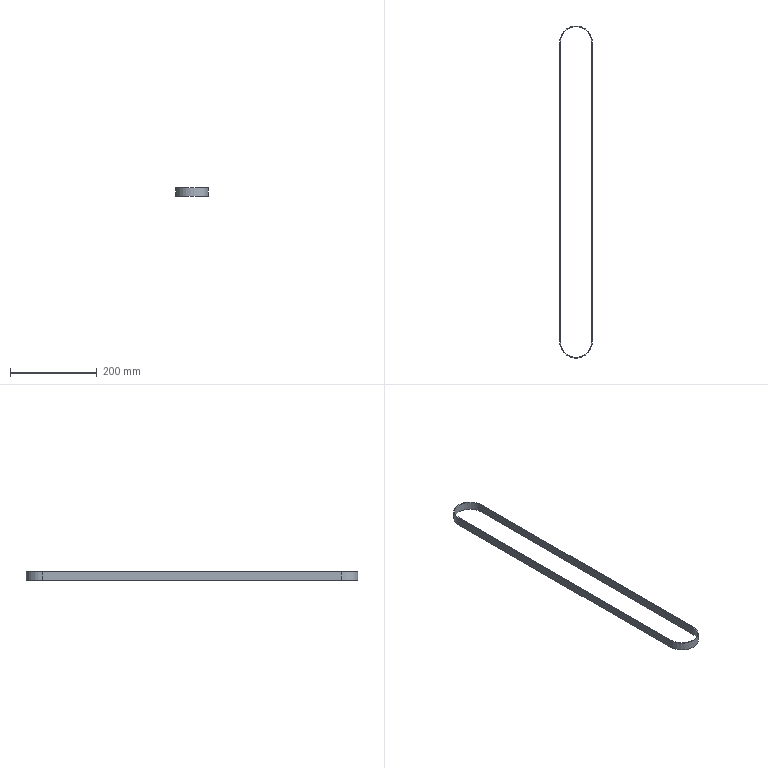Component | SolidWorks | tongbudai-1 | 1 solid | 10 faces | box 75.4 x 765.4 x 19 mm | volume 61203 mm3 | plane 6 | cylinder 4 | commonest cylinder face diameters 75.4 x2 71.4 x2
build123d program:
from build123d import *

# Parameters (mm, degrees)
EXTRUDE_THIN1_DEPTH = 9.5


with BuildPart() as part:
    # Sketch1 → Extrude-Thin1 (new, symmetric)
    with BuildSketch(Plane.XY):
        with BuildLine():
            Line((-37.7, -345), (-37.7, 345))
            ThreePointArc((-37.7, 345), (0, 382.7), (37.7, 345))
            Line((37.7, 345), (37.7, -345))
            ThreePointArc((37.7, -345), (0, -382.7), (-37.7, -345))
        make_face()
        with BuildLine():
            Line((-35.7, -345), (-35.7, 345))
            ThreePointArc((-35.7, 345), (0, 380.7), (35.7, 345))
            Line((35.7, 345), (35.7, -345))
            ThreePointArc((35.7, -345), (0, -380.7), (-35.7, -345))
        make_face(mode=Mode.SUBTRACT)
    extrude(amount=EXTRUDE_THIN1_DEPTH, both=True)


solid = part.part

# Placed as in the assembly
solid = solid.moved(Location((-25.633, -29.591, 38.5), (0, 0, 0)))
STEP:
#1=COLOUR_RGB('',0.7922,0.8196,0.9333);
#2=FILL_AREA_STYLE_COLOUR('',#1);
#3=FILL_AREA_STYLE('',(#2));
#4=SURFACE_STYLE_FILL_AREA(#3);
#5=SURFACE_SIDE_STYLE('',(#4));
#6=SURFACE_STYLE_USAGE(.BOTH.,#5);
#7=PRESENTATION_STYLE_ASSIGNMENT((#6));
#8=CARTESIAN_POINT('',(0.4751,12.418,1.89));
#9=VERTEX_POINT('',#8);
#10=CARTESIAN_POINT('',(-2.493,12.418,1.89));
#11=VERTEX_POINT('',#10);
#12=CARTESIAN_POINT('',(-1.009,12.418,1.89));
#13=DIRECTION('',(0.,0.,1.));
#14=DIRECTION('',(1.,0.,0.));
#15=AXIS2_PLACEMENT_3D('',#12,#13,#14);
#16=CIRCLE('',#15,1.484);
#17=EDGE_CURVE('',#9,#11,#16,.T.);
#18=ORIENTED_EDGE('',*,*,#17,.T.);
#19=CARTESIAN_POINT('',(-2.493,-14.748,1.89));
#20=VERTEX_POINT('',#19);
#21=CARTESIAN_POINT('',(-2.493,12.418,1.89));
#22=DIRECTION('',(0.,-1.,0.));
#23=VECTOR('',#22,39.37);
#24=LINE('',#21,#23);
#25=EDGE_CURVE('',#11,#20,#24,.T.);
#26=ORIENTED_EDGE('',*,*,#25,.T.);
#27=CARTESIAN_POINT('',(0.4751,-14.748,1.89));
#28=VERTEX_POINT('',#27);
#29=CARTESIAN_POINT('',(-1.009,-14.748,1.89));
#30=DIRECTION('',(0.,0.,1.));
#31=DIRECTION('',(1.,0.,0.));
#32=AXIS2_PLACEMENT_3D('',#29,#30,#31);
#33=CIRCLE('',#32,1.484);
#34=EDGE_CURVE('',#20,#28,#33,.T.);
#35=ORIENTED_EDGE('',*,*,#34,.T.);
#36=CARTESIAN_POINT('',(0.4751,12.418,1.89));
#37=DIRECTION('',(0.,1.,0.));
#38=VECTOR('',#37,39.37);
#39=LINE('',#36,#38);
#40=EDGE_CURVE('',#28,#9,#39,.T.);
#41=ORIENTED_EDGE('',*,*,#40,.T.);
#42=EDGE_LOOP('',(#18,#26,#35,#41));
#43=FACE_OUTER_BOUND('',#42,.T.);
#44=CARTESIAN_POINT('',(-2.415,12.418,1.89));
#45=VERTEX_POINT('',#44);
#46=CARTESIAN_POINT('',(-2.415,-14.748,1.89));
#47=VERTEX_POINT('',#46);
#48=CARTESIAN_POINT('',(-2.415,12.418,1.89));
#49=DIRECTION('',(0.,-1.,0.));
#50=VECTOR('',#49,39.37);
#51=LINE('',#48,#50);
#52=EDGE_CURVE('',#45,#47,#51,.T.);
#53=ORIENTED_EDGE('',*,*,#52,.F.);
#54=CARTESIAN_POINT('',(0.3963,12.418,1.89));
#55=VERTEX_POINT('',#54);
#56=CARTESIAN_POINT('',(-1.009,12.418,1.89));
#57=DIRECTION('',(0.,0.,1.));
#58=DIRECTION('',(1.,0.,0.));
#59=AXIS2_PLACEMENT_3D('',#56,#57,#58);
#60=CIRCLE('',#59,1.406);
#61=EDGE_CURVE('',#55,#45,#60,.T.);
#62=ORIENTED_EDGE('',*,*,#61,.F.);
#63=CARTESIAN_POINT('',(0.3963,-14.748,1.89));
#64=VERTEX_POINT('',#63);
#65=CARTESIAN_POINT('',(0.3963,12.418,1.89));
#66=DIRECTION('',(0.,1.,0.));
#67=VECTOR('',#66,39.37);
#68=LINE('',#65,#67);
#69=EDGE_CURVE('',#64,#55,#68,.T.);
#70=ORIENTED_EDGE('',*,*,#69,.F.);
#71=CARTESIAN_POINT('',(-1.009,-14.748,1.89));
#72=DIRECTION('',(0.,0.,1.));
#73=DIRECTION('',(1.,0.,0.));
#74=AXIS2_PLACEMENT_3D('',#71,#72,#73);
#75=CIRCLE('',#74,1.406);
#76=EDGE_CURVE('',#47,#64,#75,.T.);
#77=ORIENTED_EDGE('',*,*,#76,.F.);
#78=EDGE_LOOP('',(#53,#62,#70,#77));
#79=FACE_BOUND('',#78,.T.);
#80=CARTESIAN_POINT('',(-1.009,12.418,1.89));
#81=DIRECTION('',(0.,0.,1.));
#82=DIRECTION('',(1.,0.,0.));
#83=AXIS2_PLACEMENT_3D('',#80,#81,#82);
#84=PLANE('',#83);
#85=ADVANCED_FACE('',(#43,#79),#84,.T.);
#86=CARTESIAN_POINT('',(0.4751,12.418,1.142));
#87=VERTEX_POINT('',#86);
#88=CARTESIAN_POINT('',(-2.493,12.418,1.142));
#89=VERTEX_POINT('',#88);
#90=CARTESIAN_POINT('',(-1.009,12.418,1.142));
#91=DIRECTION('',(0.,0.,1.));
#92=DIRECTION('',(1.,0.,0.));
#93=AXIS2_PLACEMENT_3D('',#90,#91,#92);
#94=CIRCLE('',#93,1.484);
#95=EDGE_CURVE('',#87,#89,#94,.T.);
#96=ORIENTED_EDGE('',*,*,#95,.F.);
#97=CARTESIAN_POINT('',(0.4751,-14.748,1.142));
#98=VERTEX_POINT('',#97);
#99=CARTESIAN_POINT('',(0.4751,12.418,1.142));
#100=DIRECTION('',(0.,1.,0.));
#101=VECTOR('',#100,39.37);
#102=LINE('',#99,#101);
#103=EDGE_CURVE('',#98,#87,#102,.T.);
#104=ORIENTED_EDGE('',*,*,#103,.F.);
#105=CARTESIAN_POINT('',(-2.493,-14.748,1.142));
#106=VERTEX_POINT('',#105);
#107=CARTESIAN_POINT('',(-1.009,-14.748,1.142));
#108=DIRECTION('',(0.,0.,1.));
#109=DIRECTION('',(1.,0.,0.));
#110=AXIS2_PLACEMENT_3D('',#107,#108,#109);
#111=CIRCLE('',#110,1.484);
#112=EDGE_CURVE('',#106,#98,#111,.T.);
#113=ORIENTED_EDGE('',*,*,#112,.F.);
#114=CARTESIAN_POINT('',(-2.493,12.418,1.142));
#115=DIRECTION('',(0.,-1.,0.));
#116=VECTOR('',#115,39.37);
#117=LINE('',#114,#116);
#118=EDGE_CURVE('',#89,#106,#117,.T.);
#119=ORIENTED_EDGE('',*,*,#118,.F.);
#120=EDGE_LOOP('',(#96,#104,#113,#119));
#121=FACE_OUTER_BOUND('',#120,.T.);
#122=CARTESIAN_POINT('',(0.3963,12.418,1.142));
#123=VERTEX_POINT('',#122);
#124=CARTESIAN_POINT('',(-2.415,12.418,1.142));
#125=VERTEX_POINT('',#124);
#126=CARTESIAN_POINT('',(-1.009,12.418,1.142));
#127=DIRECTION('',(0.,0.,1.));
#128=DIRECTION('',(1.,0.,0.));
#129=AXIS2_PLACEMENT_3D('',#126,#127,#128);
#130=CIRCLE('',#129,1.406);
#131=EDGE_CURVE('',#123,#125,#130,.T.);
#132=ORIENTED_EDGE('',*,*,#131,.T.);
#133=CARTESIAN_POINT('',(-2.415,-14.748,1.142));
#134=VERTEX_POINT('',#133);
#135=CARTESIAN_POINT('',(-2.415,12.418,1.142));
#136=DIRECTION('',(0.,-1.,0.));
#137=VECTOR('',#136,39.37);
#138=LINE('',#135,#137);
#139=EDGE_CURVE('',#125,#134,#138,.T.);
#140=ORIENTED_EDGE('',*,*,#139,.T.);
#141=CARTESIAN_POINT('',(0.3963,-14.748,1.142));
#142=VERTEX_POINT('',#141);
#143=CARTESIAN_POINT('',(-1.009,-14.748,1.142));
#144=DIRECTION('',(0.,0.,1.));
#145=DIRECTION('',(1.,0.,0.));
#146=AXIS2_PLACEMENT_3D('',#143,#144,#145);
#147=CIRCLE('',#146,1.406);
#148=EDGE_CURVE('',#134,#142,#147,.T.);
#149=ORIENTED_EDGE('',*,*,#148,.T.);
#150=CARTESIAN_POINT('',(0.3963,12.418,1.142));
#151=DIRECTION('',(0.,1.,0.));
#152=VECTOR('',#151,39.37);
#153=LINE('',#150,#152);
#154=EDGE_CURVE('',#142,#123,#153,.T.);
#155=ORIENTED_EDGE('',*,*,#154,.T.);
#156=EDGE_LOOP('',(#132,#140,#149,#155));
#157=FACE_BOUND('',#156,.T.);
#158=CARTESIAN_POINT('',(-1.009,12.418,1.142));
#159=DIRECTION('',(0.,0.,1.));
#160=DIRECTION('',(1.,0.,0.));
#161=AXIS2_PLACEMENT_3D('',#158,#159,#160);
#162=PLANE('',#161);
#163=ADVANCED_FACE('',(#121,#157),#162,.F.);
#164=ORIENTED_EDGE('',*,*,#95,.T.);
#165=CARTESIAN_POINT('',(-2.493,12.418,1.89));
#166=DIRECTION('',(0.,0.,-1.));
#167=VECTOR('',#166,39.37);
#168=LINE('',#165,#167);
#169=EDGE_CURVE('',#11,#89,#168,.T.);
#170=ORIENTED_EDGE('',*,*,#169,.F.);
#171=ORIENTED_EDGE('',*,*,#17,.F.);
#172=CARTESIAN_POINT('',(0.4751,12.418,1.89));
#173=DIRECTION('',(0.,0.,-1.));
#174=VECTOR('',#173,39.37);
#175=LINE('',#172,#174);
#176=EDGE_CURVE('',#9,#87,#175,.T.);
#177=ORIENTED_EDGE('',*,*,#176,.T.);
#178=EDGE_LOOP('',(#164,#170,#171,#177));
#179=FACE_OUTER_BOUND('',#178,.T.);
#180=CARTESIAN_POINT('',(-1.009,12.418,1.89));
#181=DIRECTION('',(0.,0.,-1.));
#182=DIRECTION('',(-1.,0.,0.));
#183=AXIS2_PLACEMENT_3D('',#180,#181,#182);
#184=CYLINDRICAL_SURFACE('',#183,1.484);
#185=ADVANCED_FACE('',(#179),#184,.T.);
#186=ORIENTED_EDGE('',*,*,#118,.T.);
#187=CARTESIAN_POINT('',(-2.493,-14.748,1.89));
#188=DIRECTION('',(0.,0.,-1.));
#189=VECTOR('',#188,39.37);
#190=LINE('',#187,#189);
#191=EDGE_CURVE('',#20,#106,#190,.T.);
#192=ORIENTED_EDGE('',*,*,#191,.F.);
#193=ORIENTED_EDGE('',*,*,#25,.F.);
#194=ORIENTED_EDGE('',*,*,#169,.T.);
#195=EDGE_LOOP('',(#186,#192,#193,#194));
#196=FACE_OUTER_BOUND('',#195,.T.);
#197=CARTESIAN_POINT('',(-2.493,12.418,1.89));
#198=DIRECTION('',(1.,0.,0.));
#199=DIRECTION('',(0.,0.,-1.));
#200=AXIS2_PLACEMENT_3D('',#197,#198,#199);
#201=PLANE('',#200);
#202=ADVANCED_FACE('',(#196),#201,.F.);
#203=ORIENTED_EDGE('',*,*,#112,.T.);
#204=CARTESIAN_POINT('',(0.4751,-14.748,1.89));
#205=DIRECTION('',(0.,0.,-1.));
#206=VECTOR('',#205,39.37);
#207=LINE('',#204,#206);
#208=EDGE_CURVE('',#28,#98,#207,.T.);
#209=ORIENTED_EDGE('',*,*,#208,.F.);
#210=ORIENTED_EDGE('',*,*,#34,.F.);
#211=ORIENTED_EDGE('',*,*,#191,.T.);
#212=EDGE_LOOP('',(#203,#209,#210,#211));
#213=FACE_OUTER_BOUND('',#212,.T.);
#214=CARTESIAN_POINT('',(-1.009,-14.748,1.89));
#215=DIRECTION('',(0.,0.,-1.));
#216=DIRECTION('',(-1.,0.,0.));
#217=AXIS2_PLACEMENT_3D('',#214,#215,#216);
#218=CYLINDRICAL_SURFACE('',#217,1.484);
#219=ADVANCED_FACE('',(#213),#218,.T.);
#220=ORIENTED_EDGE('',*,*,#103,.T.);
#221=ORIENTED_EDGE('',*,*,#176,.F.);
#222=ORIENTED_EDGE('',*,*,#40,.F.);
#223=ORIENTED_EDGE('',*,*,#208,.T.);
#224=EDGE_LOOP('',(#220,#221,#222,#223));
#225=FACE_OUTER_BOUND('',#224,.T.);
#226=CARTESIAN_POINT('',(0.4751,12.418,1.89));
#227=DIRECTION('',(-1.,0.,0.));
#228=DIRECTION('',(0.,0.,1.));
#229=AXIS2_PLACEMENT_3D('',#226,#227,#228);
#230=PLANE('',#229);
#231=ADVANCED_FACE('',(#225),#230,.F.);
#232=ORIENTED_EDGE('',*,*,#131,.F.);
#233=CARTESIAN_POINT('',(0.3963,12.418,1.89));
#234=DIRECTION('',(0.,0.,-1.));
#235=VECTOR('',#234,39.37);
#236=LINE('',#233,#235);
#237=EDGE_CURVE('',#55,#123,#236,.T.);
#238=ORIENTED_EDGE('',*,*,#237,.F.);
#239=ORIENTED_EDGE('',*,*,#61,.T.);
#240=CARTESIAN_POINT('',(-2.415,12.418,1.89));
#241=DIRECTION('',(0.,0.,-1.));
#242=VECTOR('',#241,39.37);
#243=LINE('',#240,#242);
#244=EDGE_CURVE('',#45,#125,#243,.T.);
#245=ORIENTED_EDGE('',*,*,#244,.T.);
#246=EDGE_LOOP('',(#232,#238,#239,#245));
#247=FACE_OUTER_BOUND('',#246,.T.);
#248=CARTESIAN_POINT('',(-1.009,12.418,1.89));
#249=DIRECTION('',(0.,0.,-1.));
#250=DIRECTION('',(-1.,0.,0.));
#251=AXIS2_PLACEMENT_3D('',#248,#249,#250);
#252=CYLINDRICAL_SURFACE('',#251,1.406);
#253=ADVANCED_FACE('',(#247),#252,.F.);
#254=ORIENTED_EDGE('',*,*,#139,.F.);
#255=ORIENTED_EDGE('',*,*,#244,.F.);
#256=ORIENTED_EDGE('',*,*,#52,.T.);
#257=CARTESIAN_POINT('',(-2.415,-14.748,1.89));
#258=DIRECTION('',(0.,0.,-1.));
#259=VECTOR('',#258,39.37);
#260=LINE('',#257,#259);
#261=EDGE_CURVE('',#47,#134,#260,.T.);
#262=ORIENTED_EDGE('',*,*,#261,.T.);
#263=EDGE_LOOP('',(#254,#255,#256,#262));
#264=FACE_OUTER_BOUND('',#263,.T.);
#265=CARTESIAN_POINT('',(-2.415,12.418,1.89));
#266=DIRECTION('',(1.,0.,0.));
#267=DIRECTION('',(0.,0.,-1.));
#268=AXIS2_PLACEMENT_3D('',#265,#266,#267);
#269=PLANE('',#268);
#270=ADVANCED_FACE('',(#264),#269,.T.);
#271=ORIENTED_EDGE('',*,*,#148,.F.);
#272=ORIENTED_EDGE('',*,*,#261,.F.);
#273=ORIENTED_EDGE('',*,*,#76,.T.);
#274=CARTESIAN_POINT('',(0.3963,-14.748,1.89));
#275=DIRECTION('',(0.,0.,-1.));
#276=VECTOR('',#275,39.37);
#277=LINE('',#274,#276);
#278=EDGE_CURVE('',#64,#142,#277,.T.);
#279=ORIENTED_EDGE('',*,*,#278,.T.);
#280=EDGE_LOOP('',(#271,#272,#273,#279));
#281=FACE_OUTER_BOUND('',#280,.T.);
#282=CARTESIAN_POINT('',(-1.009,-14.748,1.89));
#283=DIRECTION('',(0.,0.,-1.));
#284=DIRECTION('',(-1.,0.,0.));
#285=AXIS2_PLACEMENT_3D('',#282,#283,#284);
#286=CYLINDRICAL_SURFACE('',#285,1.406);
#287=ADVANCED_FACE('',(#281),#286,.F.);
#288=ORIENTED_EDGE('',*,*,#154,.F.);
#289=ORIENTED_EDGE('',*,*,#278,.F.);
#290=ORIENTED_EDGE('',*,*,#69,.T.);
#291=ORIENTED_EDGE('',*,*,#237,.T.);
#292=EDGE_LOOP('',(#288,#289,#290,#291));
#293=FACE_OUTER_BOUND('',#292,.T.);
#294=CARTESIAN_POINT('',(0.3963,12.418,1.89));
#295=DIRECTION('',(-1.,0.,0.));
#296=DIRECTION('',(0.,0.,1.));
#297=AXIS2_PLACEMENT_3D('',#294,#295,#296);
#298=PLANE('',#297);
#299=ADVANCED_FACE('',(#293),#298,.T.);
#300=CLOSED_SHELL('',(#85,#163,#185,#202,#219,#231,#253,#270,#287,#299));
#301=MANIFOLD_SOLID_BREP('',#300);
#302=STYLED_ITEM('',(#7),#301);
#303=(LENGTH_UNIT()NAMED_UNIT(*)SI_UNIT($,.METRE.));
#304=LENGTH_MEASURE_WITH_UNIT(LENGTH_MEASURE(0.0254),#303);
#305=DIMENSIONAL_EXPONENTS(1.,0.,0.,0.,0.,0.,0.);
#306=(CONVERSION_BASED_UNIT('',#304)LENGTH_UNIT()NAMED_UNIT(#305));
#307=UNCERTAINTY_MEASURE_WITH_UNIT(LENGTH_MEASURE(0.00001),#306,'','');
#308=(NAMED_UNIT(*)PLANE_ANGLE_UNIT()SI_UNIT($,.RADIAN.));
#309=(NAMED_UNIT(*)SI_UNIT($,.STERADIAN.)SOLID_ANGLE_UNIT());
#310=(GEOMETRIC_REPRESENTATION_CONTEXT(3)GLOBAL_UNCERTAINTY_ASSIGNED_CONTEXT((#307))GLOBAL_UNIT_ASSIGNED_CONTEXT((#306,#308,#309))REPRESENTATION_CONTEXT('',''));
#311=MECHANICAL_DESIGN_GEOMETRIC_PRESENTATION_REPRESENTATION('',(#302),#310);
#312=PRESENTATION_LAYER_ASSIGNMENT('','',(#302));
#313=CARTESIAN_POINT('',(0.,0.,0.));
#314=DIRECTION('',(0.,0.,1.));
#315=DIRECTION('',(1.,0.,0.));
#316=AXIS2_PLACEMENT_3D('',#313,#314,#315);
#317=(LENGTH_UNIT()NAMED_UNIT(*)SI_UNIT($,.METRE.));
#318=LENGTH_MEASURE_WITH_UNIT(LENGTH_MEASURE(0.0254),#317);
#319=DIMENSIONAL_EXPONENTS(1.,0.,0.,0.,0.,0.,0.);
#320=(CONVERSION_BASED_UNIT('',#318)LENGTH_UNIT()NAMED_UNIT(#319));
#321=UNCERTAINTY_MEASURE_WITH_UNIT(LENGTH_MEASURE(0.00001),#320,'','');
#322=(NAMED_UNIT(*)PLANE_ANGLE_UNIT()SI_UNIT($,.RADIAN.));
#323=(NAMED_UNIT(*)SI_UNIT($,.STERADIAN.)SOLID_ANGLE_UNIT());
#324=(GEOMETRIC_REPRESENTATION_CONTEXT(3)GLOBAL_UNCERTAINTY_ASSIGNED_CONTEXT((#321))GLOBAL_UNIT_ASSIGNED_CONTEXT((#320,#322,#323))REPRESENTATION_CONTEXT('',''));
#325=ADVANCED_BREP_SHAPE_REPRESENTATION('',(#301,#316),#324);